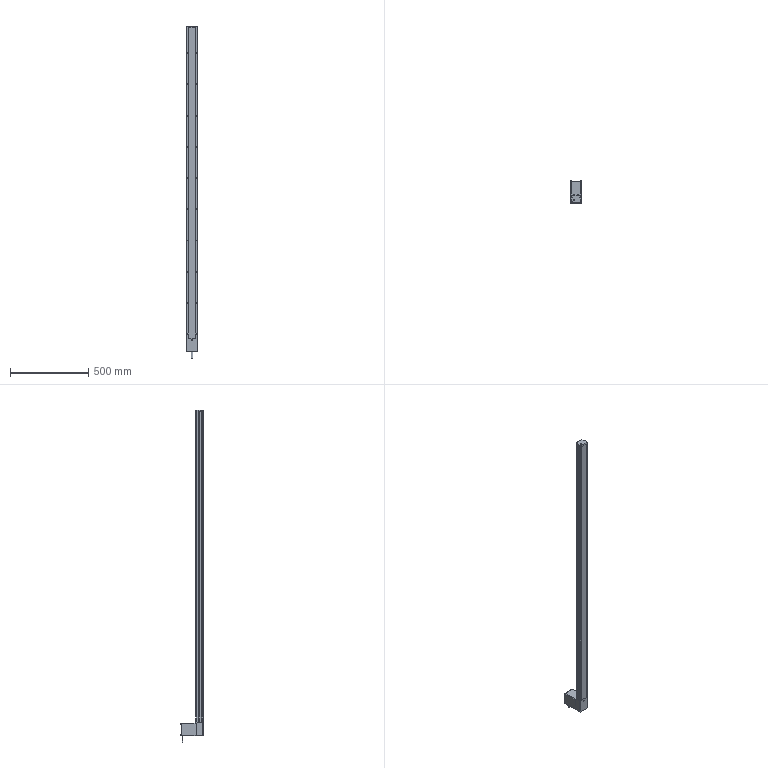Component | SolidWorks | LEFB32T-1800(0_0_0)-1_LEFB32T-1800(0_0_0)1-1 | 1 solid | 240 faces | volume 6392546 mm3 | cylinder 110 | plane 110 | spline 16 | cone 4 | commonest cylinder face diameters 5.5 x42 5.6 x16 4 x16 6 x14 2 x8 5 x6 7 x6 3.242 x2